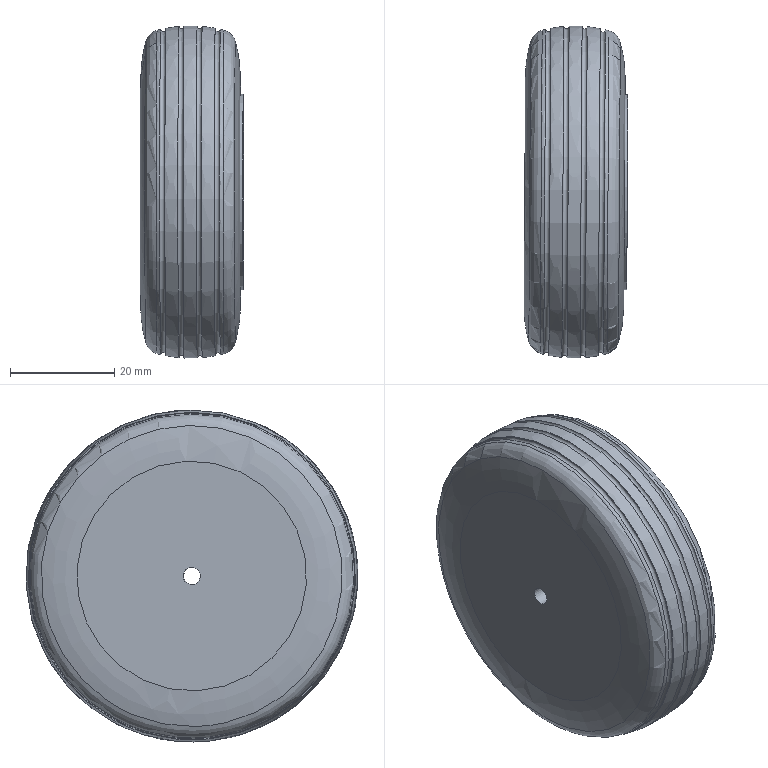Component | NX | WHEEL | 1 solid | 26 faces | volume 53472 mm3 | plane 8 | spline 7 | torus 7 | cylinder 4 | commonest cylinder face diameters 37.522 x1 34.412 x1 6.35 x1 3.3 x1